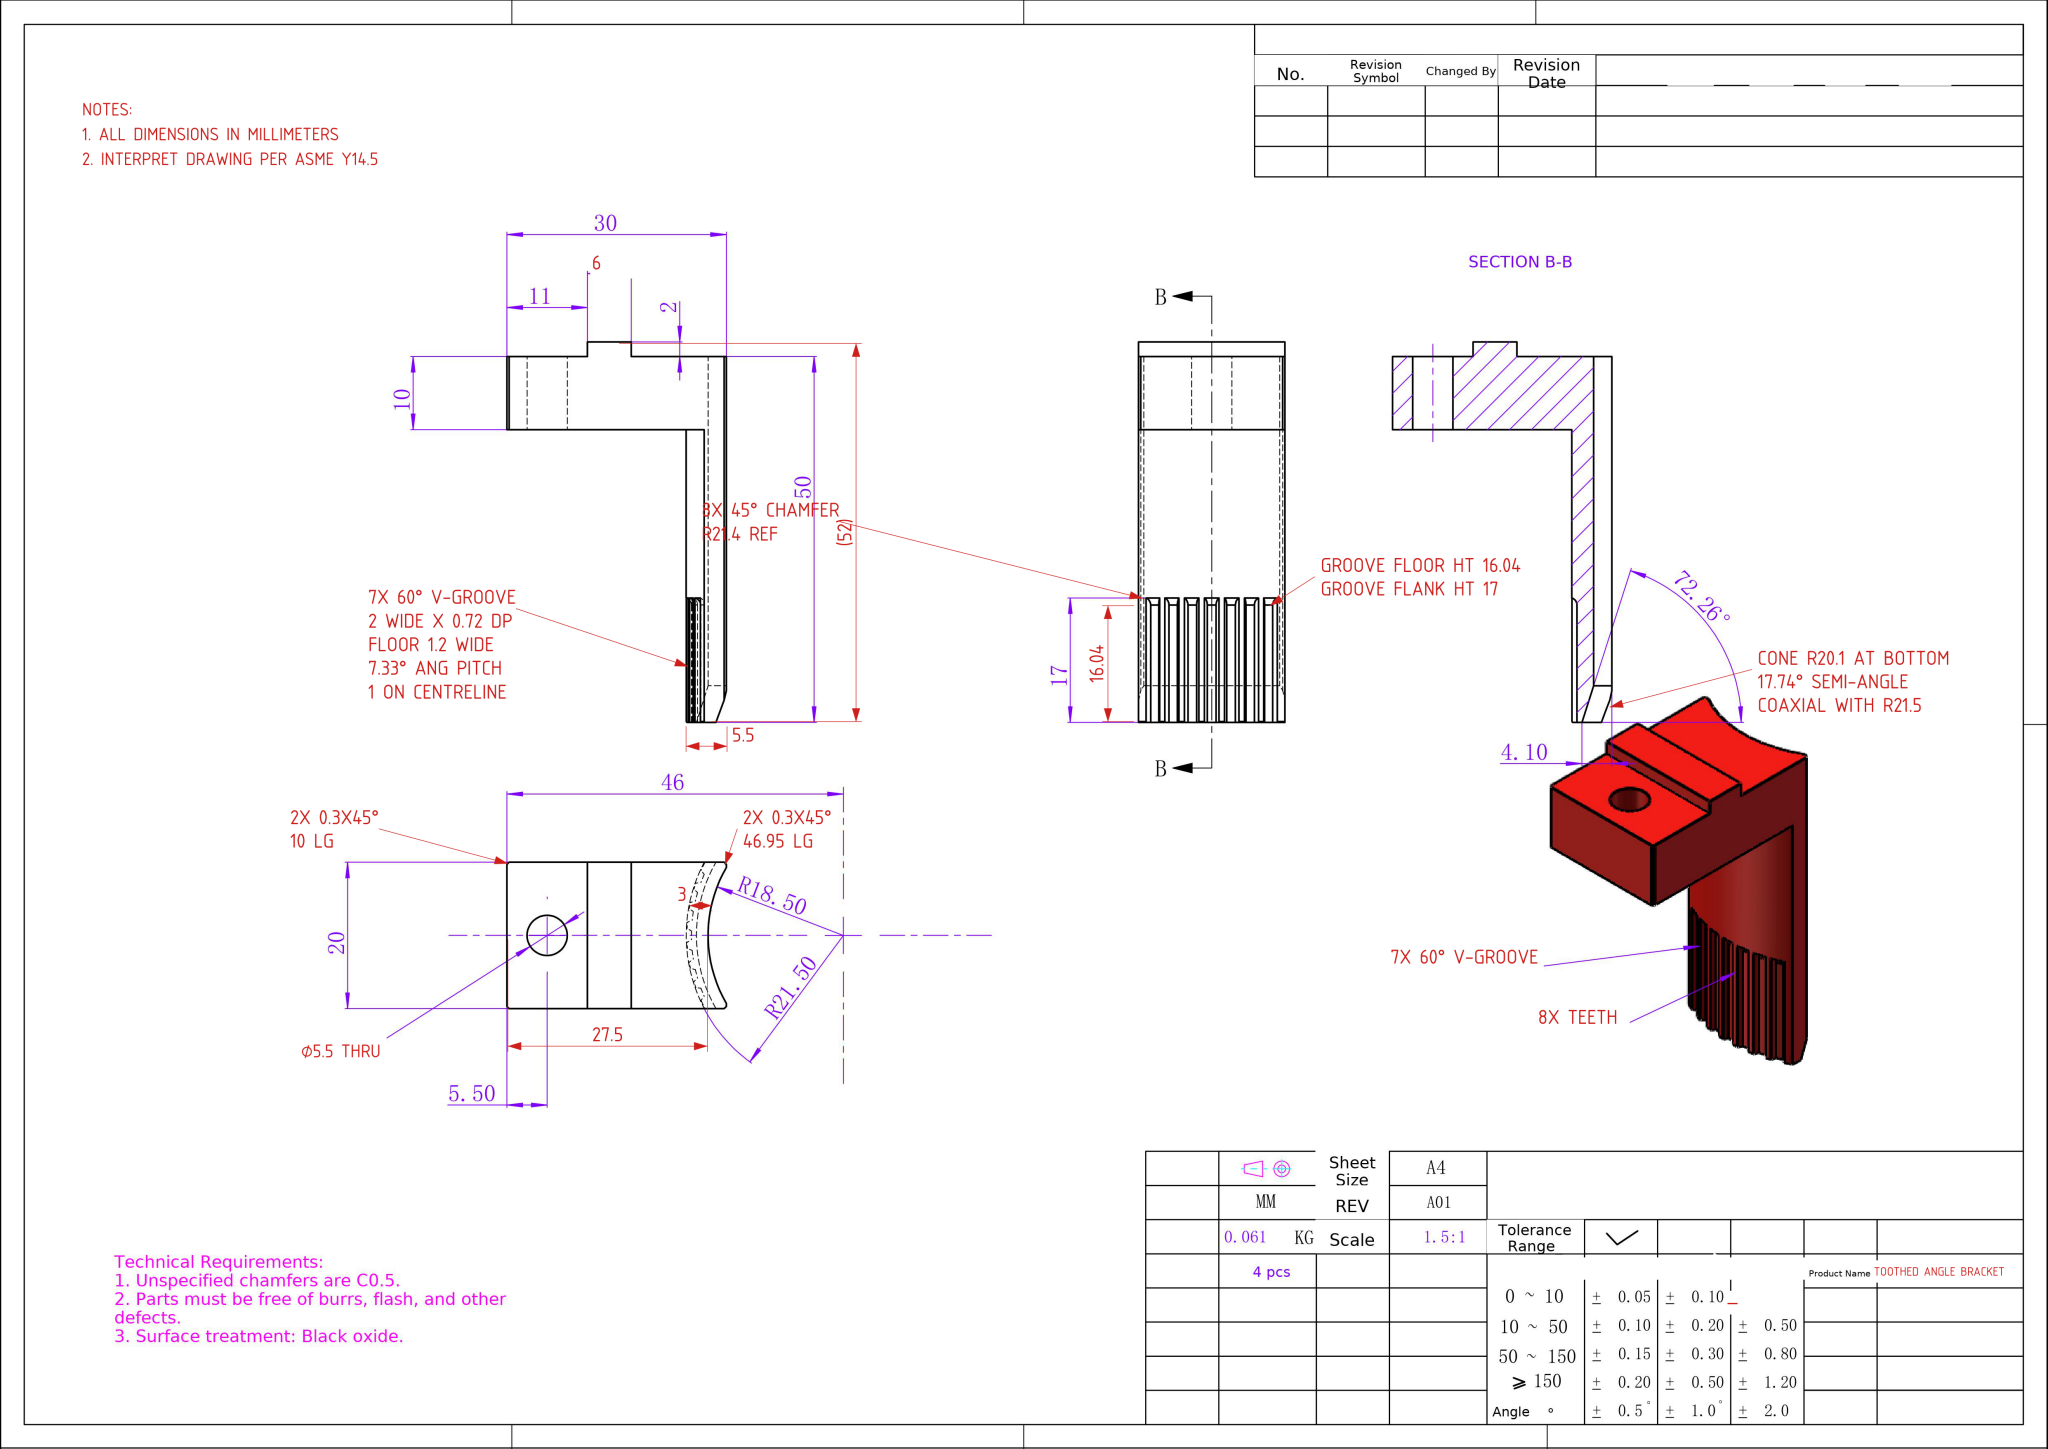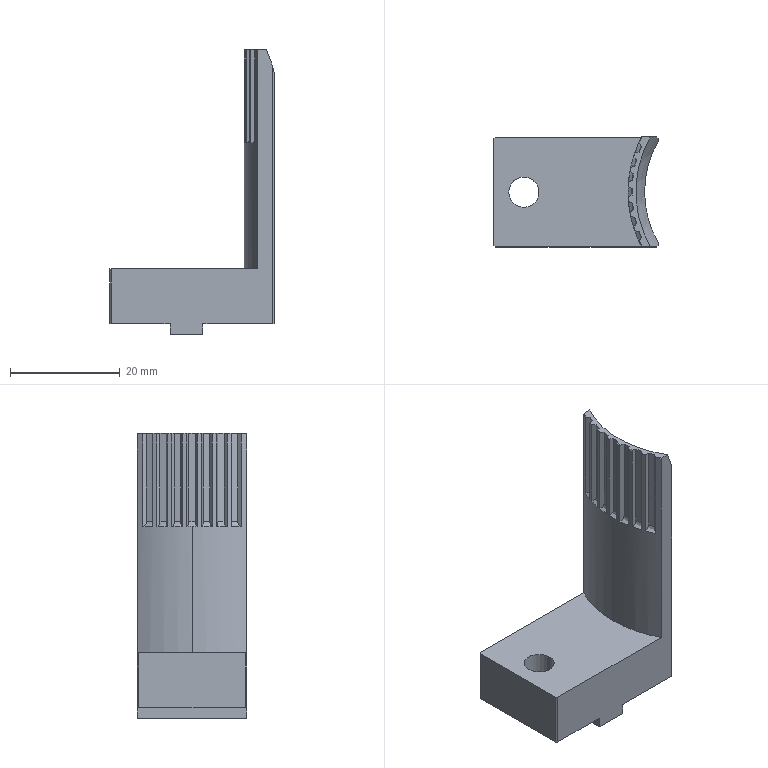Part | NX | mm | 1 solid | 59 faces | box 30 x 20 x 52 mm | volume 7968 mm3 | plane 37 | cone 9 | spline 7 | cylinder 6 | commonest cylinder face diameters 5.5 x2 43 x2 37 x2